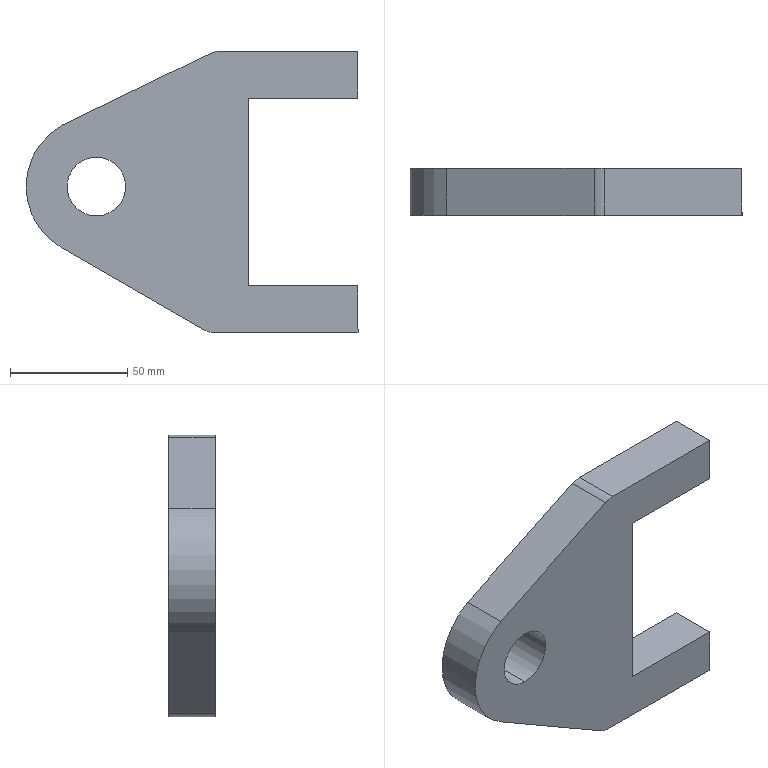Component | SolidWorks | 7TractionPlate-2 | 1 solid | 16 faces | box 141.51 x 20 x 120 mm | volume 186716 mm3 | plane 11 | cylinder 5 | commonest cylinder face diameters 25 x2 20 x2 60 x1
build123d program:
from build123d import *

# Parameters (mm, degrees)
SKETCH1_R           = 12.5
BOSS_EXTRUDE1_DEPTH = 20


with BuildPart() as part:
    # Sketch1 → Boss-Extrude1 (new body)
    with BuildSketch(Plane.XY):
        with BuildLine():
            Line((-34.563, 94.573), (-69.563, 33.951))
            ThreePointArc((-69.563, 33.951), (-70.562, 31.539), (-70.903, 28.951))
            Line((-70.903, 28.951), (-70.903, -31.936))
            Line((-70.903, -31.936), (-50.903, -31.936))
            Line((-50.903, -31.936), (-50.903, 14.622))
            Line((-50.903, 14.622), (29.097, 14.622))
            Line((29.097, 14.622), (29.097, -31.936))
            Line((29.097, -31.936), (40, -31.936))
            Line((40, -31.936), (49.097, -31.936))
            Line((49.097, -31.936), (49.097, 26.72))
            ThreePointArc((49.097, 26.72), (48.845, 28.95), (48.102, 31.068))
            Line((48.102, 31.068), (17.664, 94.104))
            ThreePointArc((17.664, 94.104), (-8.313, 109.571), (-34.563, 94.573))
        make_face()
        with Locations((-8.582, 79.573)):
            Circle(SKETCH1_R, mode=Mode.SUBTRACT)
    extrude(amount=BOSS_EXTRUDE1_DEPTH)


solid = part.part

# Placed as in the assembly
solid = solid.moved(Location((213.102, -253.79, 608.582), (90, 0, 90)))
STEP:
#1=COLOUR_RGB('',0.7922,0.8196,0.9333);
#2=FILL_AREA_STYLE_COLOUR('',#1);
#3=FILL_AREA_STYLE('',(#2));
#4=SURFACE_STYLE_FILL_AREA(#3);
#5=SURFACE_SIDE_STYLE('',(#4));
#6=SURFACE_STYLE_USAGE(.BOTH.,#5);
#7=PRESENTATION_STYLE_ASSIGNMENT((#6));
#8=CARTESIAN_POINT('',(5.257,-10.779,23.13));
#9=VERTEX_POINT('',#8);
#10=CARTESIAN_POINT('',(5.257,-10.779,24.114));
#11=VERTEX_POINT('',#10);
#12=CARTESIAN_POINT('',(5.257,-10.779,23.622));
#13=DIRECTION('',(0.,-1.,0.));
#14=DIRECTION('',(-0.,0.,1.));
#15=AXIS2_PLACEMENT_3D('',#12,#13,#14);
#16=CIRCLE('',#15,0.4921);
#17=EDGE_CURVE('',#9,#11,#16,.T.);
#18=ORIENTED_EDGE('',*,*,#17,.T.);
#19=CARTESIAN_POINT('',(5.257,-9.992,24.114));
#20=VERTEX_POINT('',#19);
#21=CARTESIAN_POINT('',(5.257,-10.779,24.114));
#22=DIRECTION('',(-0.,1.,-0.));
#23=VECTOR('',#22,39.37);
#24=LINE('',#21,#23);
#25=EDGE_CURVE('',#11,#20,#24,.T.);
#26=ORIENTED_EDGE('',*,*,#25,.T.);
#27=CARTESIAN_POINT('',(5.257,-9.992,23.13));
#28=VERTEX_POINT('',#27);
#29=CARTESIAN_POINT('',(5.257,-9.992,23.622));
#30=DIRECTION('',(0.,-1.,0.));
#31=DIRECTION('',(-0.,0.,1.));
#32=AXIS2_PLACEMENT_3D('',#29,#30,#31);
#33=CIRCLE('',#32,0.4921);
#34=EDGE_CURVE('',#28,#20,#33,.T.);
#35=ORIENTED_EDGE('',*,*,#34,.F.);
#36=CARTESIAN_POINT('',(5.257,-10.779,23.13));
#37=DIRECTION('',(-0.,1.,-0.));
#38=VECTOR('',#37,39.37);
#39=LINE('',#36,#38);
#40=EDGE_CURVE('',#9,#28,#39,.T.);
#41=ORIENTED_EDGE('',*,*,#40,.F.);
#42=EDGE_LOOP('',(#18,#26,#35,#41));
#43=FACE_OUTER_BOUND('',#42,.T.);
#44=CARTESIAN_POINT('',(5.257,-10.779,23.622));
#45=DIRECTION('',(-0.,1.,-0.));
#46=DIRECTION('',(0.,-0.,-1.));
#47=AXIS2_PLACEMENT_3D('',#44,#45,#46);
#48=CYLINDRICAL_SURFACE('',#47,0.4921);
#49=ADVANCED_FACE('',(#43),#48,.F.);
#50=CARTESIAN_POINT('',(7.25,-9.992,21.168));
#51=VERTEX_POINT('',#50);
#52=CARTESIAN_POINT('',(7.053,-9.992,21.221));
#53=VERTEX_POINT('',#52);
#54=CARTESIAN_POINT('',(7.25,-9.992,21.562));
#55=DIRECTION('',(-0.,1.,-0.));
#56=DIRECTION('',(-0.,0.,1.));
#57=AXIS2_PLACEMENT_3D('',#54,#55,#56);
#58=CIRCLE('',#57,0.3937);
#59=EDGE_CURVE('',#51,#53,#58,.T.);
#60=ORIENTED_EDGE('',*,*,#59,.F.);
#61=CARTESIAN_POINT('',(7.25,-10.779,21.168));
#62=VERTEX_POINT('',#61);
#63=CARTESIAN_POINT('',(7.25,-10.779,21.168));
#64=DIRECTION('',(-0.,1.,-0.));
#65=VECTOR('',#64,39.37);
#66=LINE('',#63,#65);
#67=EDGE_CURVE('',#62,#51,#66,.T.);
#68=ORIENTED_EDGE('',*,*,#67,.F.);
#69=CARTESIAN_POINT('',(7.053,-10.779,21.221));
#70=VERTEX_POINT('',#69);
#71=CARTESIAN_POINT('',(7.25,-10.779,21.562));
#72=DIRECTION('',(-0.,1.,-0.));
#73=DIRECTION('',(0.,0.,1.));
#74=AXIS2_PLACEMENT_3D('',#71,#72,#73);
#75=CIRCLE('',#74,0.3937);
#76=EDGE_CURVE('',#62,#70,#75,.T.);
#77=ORIENTED_EDGE('',*,*,#76,.T.);
#78=CARTESIAN_POINT('',(7.053,-10.779,21.221));
#79=DIRECTION('',(-0.,1.,-0.));
#80=VECTOR('',#79,39.37);
#81=LINE('',#78,#80);
#82=EDGE_CURVE('',#70,#53,#81,.T.);
#83=ORIENTED_EDGE('',*,*,#82,.T.);
#84=EDGE_LOOP('',(#60,#68,#77,#83));
#85=FACE_OUTER_BOUND('',#84,.T.);
#86=CARTESIAN_POINT('',(7.25,-10.779,21.562));
#87=DIRECTION('',(-0.,1.,-0.));
#88=DIRECTION('',(0.,-0.,-1.));
#89=AXIS2_PLACEMENT_3D('',#86,#87,#88);
#90=CYLINDRICAL_SURFACE('',#89,0.3937);
#91=ADVANCED_FACE('',(#85),#90,.T.);
#92=CARTESIAN_POINT('',(9.647,-9.992,21.168));
#93=VERTEX_POINT('',#92);
#94=CARTESIAN_POINT('',(8.39,-9.992,21.168));
#95=DIRECTION('',(1.,0.,0.));
#96=VECTOR('',#95,39.37);
#97=LINE('',#94,#96);
#98=EDGE_CURVE('',#51,#93,#97,.T.);
#99=ORIENTED_EDGE('',*,*,#98,.T.);
#100=CARTESIAN_POINT('',(9.647,-10.779,21.168));
#101=VERTEX_POINT('',#100);
#102=CARTESIAN_POINT('',(9.647,-10.779,21.168));
#103=DIRECTION('',(-0.,1.,-0.));
#104=VECTOR('',#103,39.37);
#105=LINE('',#102,#104);
#106=EDGE_CURVE('',#101,#93,#105,.T.);
#107=ORIENTED_EDGE('',*,*,#106,.F.);
#108=CARTESIAN_POINT('',(8.39,-10.779,21.168));
#109=DIRECTION('',(1.,0.,0.));
#110=VECTOR('',#109,39.37);
#111=LINE('',#108,#110);
#112=EDGE_CURVE('',#62,#101,#111,.T.);
#113=ORIENTED_EDGE('',*,*,#112,.F.);
#114=ORIENTED_EDGE('',*,*,#67,.T.);
#115=EDGE_LOOP('',(#99,#107,#113,#114));
#116=FACE_OUTER_BOUND('',#115,.T.);
#117=CARTESIAN_POINT('',(8.39,-10.779,21.168));
#118=DIRECTION('',(-0.,0.,1.));
#119=DIRECTION('',(-1.,-0.,-0.));
#120=AXIS2_PLACEMENT_3D('',#117,#118,#119);
#121=PLANE('',#120);
#122=ADVANCED_FACE('',(#116),#121,.F.);
#123=CARTESIAN_POINT('',(9.647,-9.992,21.956));
#124=VERTEX_POINT('',#123);
#125=CARTESIAN_POINT('',(9.647,-9.992,23.96));
#126=DIRECTION('',(-0.,0.,1.));
#127=VECTOR('',#126,39.37);
#128=LINE('',#125,#127);
#129=EDGE_CURVE('',#93,#124,#128,.T.);
#130=ORIENTED_EDGE('',*,*,#129,.T.);
#131=CARTESIAN_POINT('',(9.647,-10.779,21.956));
#132=VERTEX_POINT('',#131);
#133=CARTESIAN_POINT('',(9.647,-10.779,21.956));
#134=DIRECTION('',(-0.,1.,-0.));
#135=VECTOR('',#134,39.37);
#136=LINE('',#133,#135);
#137=EDGE_CURVE('',#132,#124,#136,.T.);
#138=ORIENTED_EDGE('',*,*,#137,.F.);
#139=CARTESIAN_POINT('',(9.647,-10.779,23.96));
#140=DIRECTION('',(-0.,0.,1.));
#141=VECTOR('',#140,39.37);
#142=LINE('',#139,#141);
#143=EDGE_CURVE('',#101,#132,#142,.T.);
#144=ORIENTED_EDGE('',*,*,#143,.F.);
#145=ORIENTED_EDGE('',*,*,#106,.T.);
#146=EDGE_LOOP('',(#130,#138,#144,#145));
#147=FACE_OUTER_BOUND('',#146,.T.);
#148=CARTESIAN_POINT('',(9.647,-10.779,23.96));
#149=DIRECTION('',(-1.,-0.,-0.));
#150=DIRECTION('',(0.,-1.,0.));
#151=AXIS2_PLACEMENT_3D('',#148,#149,#150);
#152=PLANE('',#151);
#153=ADVANCED_FACE('',(#147),#152,.F.);
#154=CARTESIAN_POINT('',(7.814,-9.992,21.956));
#155=VERTEX_POINT('',#154);
#156=CARTESIAN_POINT('',(8.39,-9.992,21.956));
#157=DIRECTION('',(-1.,-0.,-0.));
#158=VECTOR('',#157,39.37);
#159=LINE('',#156,#158);
#160=EDGE_CURVE('',#124,#155,#159,.T.);
#161=ORIENTED_EDGE('',*,*,#160,.T.);
#162=CARTESIAN_POINT('',(7.814,-10.779,21.956));
#163=VERTEX_POINT('',#162);
#164=CARTESIAN_POINT('',(7.814,-10.779,21.956));
#165=DIRECTION('',(-0.,1.,-0.));
#166=VECTOR('',#165,39.37);
#167=LINE('',#164,#166);
#168=EDGE_CURVE('',#163,#155,#167,.T.);
#169=ORIENTED_EDGE('',*,*,#168,.F.);
#170=CARTESIAN_POINT('',(8.39,-10.779,21.956));
#171=DIRECTION('',(-1.,-0.,-0.));
#172=VECTOR('',#171,39.37);
#173=LINE('',#170,#172);
#174=EDGE_CURVE('',#132,#163,#173,.T.);
#175=ORIENTED_EDGE('',*,*,#174,.F.);
#176=ORIENTED_EDGE('',*,*,#137,.T.);
#177=EDGE_LOOP('',(#161,#169,#175,#176));
#178=FACE_OUTER_BOUND('',#177,.T.);
#179=CARTESIAN_POINT('',(8.39,-10.779,21.956));
#180=DIRECTION('',(0.,-0.,-1.));
#181=DIRECTION('',(0.,-1.,0.));
#182=AXIS2_PLACEMENT_3D('',#179,#180,#181);
#183=PLANE('',#182);
#184=ADVANCED_FACE('',(#178),#183,.F.);
#185=CARTESIAN_POINT('',(7.814,-9.992,25.105));
#186=VERTEX_POINT('',#185);
#187=CARTESIAN_POINT('',(7.814,-9.992,23.96));
#188=DIRECTION('',(-0.,0.,1.));
#189=VECTOR('',#188,39.37);
#190=LINE('',#187,#189);
#191=EDGE_CURVE('',#155,#186,#190,.T.);
#192=ORIENTED_EDGE('',*,*,#191,.T.);
#193=CARTESIAN_POINT('',(7.814,-10.779,25.105));
#194=VERTEX_POINT('',#193);
#195=CARTESIAN_POINT('',(7.814,-10.779,25.105));
#196=DIRECTION('',(-0.,1.,-0.));
#197=VECTOR('',#196,39.37);
#198=LINE('',#195,#197);
#199=EDGE_CURVE('',#194,#186,#198,.T.);
#200=ORIENTED_EDGE('',*,*,#199,.F.);
#201=CARTESIAN_POINT('',(7.814,-10.779,23.96));
#202=DIRECTION('',(-0.,0.,1.));
#203=VECTOR('',#202,39.37);
#204=LINE('',#201,#203);
#205=EDGE_CURVE('',#163,#194,#204,.T.);
#206=ORIENTED_EDGE('',*,*,#205,.F.);
#207=ORIENTED_EDGE('',*,*,#168,.T.);
#208=EDGE_LOOP('',(#192,#200,#206,#207));
#209=FACE_OUTER_BOUND('',#208,.T.);
#210=CARTESIAN_POINT('',(7.814,-10.779,23.96));
#211=DIRECTION('',(-1.,-0.,-0.));
#212=DIRECTION('',(0.,-1.,0.));
#213=AXIS2_PLACEMENT_3D('',#210,#211,#212);
#214=PLANE('',#213);
#215=ADVANCED_FACE('',(#209),#214,.F.);
#216=CARTESIAN_POINT('',(9.647,-9.992,25.105));
#217=VERTEX_POINT('',#216);
#218=CARTESIAN_POINT('',(8.39,-9.992,25.105));
#219=DIRECTION('',(1.,0.,0.));
#220=VECTOR('',#219,39.37);
#221=LINE('',#218,#220);
#222=EDGE_CURVE('',#186,#217,#221,.T.);
#223=ORIENTED_EDGE('',*,*,#222,.T.);
#224=CARTESIAN_POINT('',(9.647,-10.779,25.105));
#225=VERTEX_POINT('',#224);
#226=CARTESIAN_POINT('',(9.647,-10.779,25.105));
#227=DIRECTION('',(-0.,1.,-0.));
#228=VECTOR('',#227,39.37);
#229=LINE('',#226,#228);
#230=EDGE_CURVE('',#225,#217,#229,.T.);
#231=ORIENTED_EDGE('',*,*,#230,.F.);
#232=CARTESIAN_POINT('',(8.39,-10.779,25.105));
#233=DIRECTION('',(1.,0.,0.));
#234=VECTOR('',#233,39.37);
#235=LINE('',#232,#234);
#236=EDGE_CURVE('',#194,#225,#235,.T.);
#237=ORIENTED_EDGE('',*,*,#236,.F.);
#238=ORIENTED_EDGE('',*,*,#199,.T.);
#239=EDGE_LOOP('',(#223,#231,#237,#238));
#240=FACE_OUTER_BOUND('',#239,.T.);
#241=CARTESIAN_POINT('',(8.39,-10.779,25.105));
#242=DIRECTION('',(-0.,0.,1.));
#243=DIRECTION('',(-0.,1.,-0.));
#244=AXIS2_PLACEMENT_3D('',#241,#242,#243);
#245=PLANE('',#244);
#246=ADVANCED_FACE('',(#240),#245,.F.);
#247=CARTESIAN_POINT('',(9.647,-9.992,25.893));
#248=VERTEX_POINT('',#247);
#249=CARTESIAN_POINT('',(9.647,-9.992,23.96));
#250=DIRECTION('',(-0.,0.,1.));
#251=VECTOR('',#250,39.37);
#252=LINE('',#249,#251);
#253=EDGE_CURVE('',#217,#248,#252,.T.);
#254=ORIENTED_EDGE('',*,*,#253,.T.);
#255=CARTESIAN_POINT('',(9.647,-10.779,25.893));
#256=VERTEX_POINT('',#255);
#257=CARTESIAN_POINT('',(9.647,-10.779,25.893));
#258=DIRECTION('',(-0.,1.,-0.));
#259=VECTOR('',#258,39.37);
#260=LINE('',#257,#259);
#261=EDGE_CURVE('',#256,#248,#260,.T.);
#262=ORIENTED_EDGE('',*,*,#261,.F.);
#263=CARTESIAN_POINT('',(9.647,-10.779,23.96));
#264=DIRECTION('',(-0.,0.,1.));
#265=VECTOR('',#264,39.37);
#266=LINE('',#263,#265);
#267=EDGE_CURVE('',#225,#256,#266,.T.);
#268=ORIENTED_EDGE('',*,*,#267,.F.);
#269=ORIENTED_EDGE('',*,*,#230,.T.);
#270=EDGE_LOOP('',(#254,#262,#268,#269));
#271=FACE_OUTER_BOUND('',#270,.T.);
#272=CARTESIAN_POINT('',(9.647,-10.779,23.96));
#273=DIRECTION('',(-1.,-0.,-0.));
#274=DIRECTION('',(0.,-0.,-1.));
#275=AXIS2_PLACEMENT_3D('',#272,#273,#274);
#276=PLANE('',#275);
#277=ADVANCED_FACE('',(#271),#276,.F.);
#278=CARTESIAN_POINT('',(7.338,-9.992,25.893));
#279=VERTEX_POINT('',#278);
#280=CARTESIAN_POINT('',(8.39,-9.992,25.893));
#281=DIRECTION('',(1.,0.,0.));
#282=VECTOR('',#281,39.37);
#283=LINE('',#280,#282);
#284=EDGE_CURVE('',#279,#248,#283,.T.);
#285=ORIENTED_EDGE('',*,*,#284,.F.);
#286=CARTESIAN_POINT('',(7.338,-10.779,25.893));
#287=VERTEX_POINT('',#286);
#288=CARTESIAN_POINT('',(7.338,-10.779,25.893));
#289=DIRECTION('',(-0.,1.,-0.));
#290=VECTOR('',#289,39.37);
#291=LINE('',#288,#290);
#292=EDGE_CURVE('',#287,#279,#291,.T.);
#293=ORIENTED_EDGE('',*,*,#292,.F.);
#294=CARTESIAN_POINT('',(8.39,-10.779,25.893));
#295=DIRECTION('',(1.,0.,0.));
#296=VECTOR('',#295,39.37);
#297=LINE('',#294,#296);
#298=EDGE_CURVE('',#287,#256,#297,.T.);
#299=ORIENTED_EDGE('',*,*,#298,.T.);
#300=ORIENTED_EDGE('',*,*,#261,.T.);
#301=EDGE_LOOP('',(#285,#293,#299,#300));
#302=FACE_OUTER_BOUND('',#301,.T.);
#303=CARTESIAN_POINT('',(8.39,-10.779,25.893));
#304=DIRECTION('',(-0.,0.,1.));
#305=DIRECTION('',(-1.,-0.,-0.));
#306=AXIS2_PLACEMENT_3D('',#303,#304,#305);
#307=PLANE('',#306);
#308=ADVANCED_FACE('',(#302),#307,.T.);
#309=CARTESIAN_POINT('',(7.167,-9.992,25.854));
#310=VERTEX_POINT('',#309);
#311=CARTESIAN_POINT('',(7.338,-9.992,25.499));
#312=DIRECTION('',(0.,-1.,0.));
#313=DIRECTION('',(-0.,0.,1.));
#314=AXIS2_PLACEMENT_3D('',#311,#312,#313);
#315=CIRCLE('',#314,0.3937);
#316=EDGE_CURVE('',#279,#310,#315,.T.);
#317=ORIENTED_EDGE('',*,*,#316,.T.);
#318=CARTESIAN_POINT('',(7.167,-10.779,25.854));
#319=VERTEX_POINT('',#318);
#320=CARTESIAN_POINT('',(7.167,-10.779,25.854));
#321=DIRECTION('',(-0.,1.,-0.));
#322=VECTOR('',#321,39.37);
#323=LINE('',#320,#322);
#324=EDGE_CURVE('',#319,#310,#323,.T.);
#325=ORIENTED_EDGE('',*,*,#324,.F.);
#326=CARTESIAN_POINT('',(7.338,-10.779,25.499));
#327=DIRECTION('',(0.,-1.,0.));
#328=DIRECTION('',(-0.,0.,1.));
#329=AXIS2_PLACEMENT_3D('',#326,#327,#328);
#330=CIRCLE('',#329,0.3937);
#331=EDGE_CURVE('',#287,#319,#330,.T.);
#332=ORIENTED_EDGE('',*,*,#331,.F.);
#333=ORIENTED_EDGE('',*,*,#292,.T.);
#334=EDGE_LOOP('',(#317,#325,#332,#333));
#335=FACE_OUTER_BOUND('',#334,.T.);
#336=CARTESIAN_POINT('',(7.338,-10.779,25.499));
#337=DIRECTION('',(-0.,1.,-0.));
#338=DIRECTION('',(0.,-0.,-1.));
#339=AXIS2_PLACEMENT_3D('',#336,#337,#338);
#340=CYLINDRICAL_SURFACE('',#339,0.3937);
#341=ADVANCED_FACE('',(#335),#340,.T.);
#342=CARTESIAN_POINT('',(4.685,-9.992,24.655));
#343=VERTEX_POINT('',#342);
#344=CARTESIAN_POINT('',(7.417,-9.992,25.975));
#345=DIRECTION('',(0.9005,0.,0.4348));
#346=VECTOR('',#345,39.37);
#347=LINE('',#344,#346);
#348=EDGE_CURVE('',#343,#310,#347,.T.);
#349=ORIENTED_EDGE('',*,*,#348,.F.);
#350=CARTESIAN_POINT('',(4.685,-10.779,24.655));
#351=VERTEX_POINT('',#350);
#352=CARTESIAN_POINT('',(4.685,-10.779,24.655));
#353=DIRECTION('',(-0.,1.,-0.));
#354=VECTOR('',#353,39.37);
#355=LINE('',#352,#354);
#356=EDGE_CURVE('',#351,#343,#355,.T.);
#357=ORIENTED_EDGE('',*,*,#356,.F.);
#358=CARTESIAN_POINT('',(7.417,-10.779,25.975));
#359=DIRECTION('',(0.9005,0.,0.4348));
#360=VECTOR('',#359,39.37);
#361=LINE('',#358,#360);
#362=EDGE_CURVE('',#351,#319,#361,.T.);
#363=ORIENTED_EDGE('',*,*,#362,.T.);
#364=ORIENTED_EDGE('',*,*,#324,.T.);
#365=EDGE_LOOP('',(#349,#357,#363,#364));
#366=FACE_OUTER_BOUND('',#365,.T.);
#367=CARTESIAN_POINT('',(7.417,-10.779,25.975));
#368=DIRECTION('',(-0.4348,0.,0.9005));
#369=DIRECTION('',(-0.9005,-0.,-0.4348));
#370=AXIS2_PLACEMENT_3D('',#367,#368,#369);
#371=PLANE('',#370);
#372=ADVANCED_FACE('',(#366),#371,.T.);
#373=CARTESIAN_POINT('',(4.667,-9.992,22.599));
#374=VERTEX_POINT('',#373);
#375=CARTESIAN_POINT('',(5.257,-9.992,23.622));
#376=DIRECTION('',(-0.,1.,-0.));
#377=DIRECTION('',(-0.,0.,1.));
#378=AXIS2_PLACEMENT_3D('',#375,#376,#377);
#379=CIRCLE('',#378,1.181);
#380=EDGE_CURVE('',#374,#343,#379,.T.);
#381=ORIENTED_EDGE('',*,*,#380,.F.);
#382=CARTESIAN_POINT('',(4.667,-10.779,22.599));
#383=VERTEX_POINT('',#382);
#384=CARTESIAN_POINT('',(4.667,-10.779,22.599));
#385=DIRECTION('',(-0.,1.,-0.));
#386=VECTOR('',#385,39.37);
#387=LINE('',#384,#386);
#388=EDGE_CURVE('',#383,#374,#387,.T.);
#389=ORIENTED_EDGE('',*,*,#388,.F.);
#390=CARTESIAN_POINT('',(5.257,-10.779,23.622));
#391=DIRECTION('',(-0.,1.,-0.));
#392=DIRECTION('',(-0.,0.,1.));
#393=AXIS2_PLACEMENT_3D('',#390,#391,#392);
#394=CIRCLE('',#393,1.181);
#395=EDGE_CURVE('',#383,#351,#394,.T.);
#396=ORIENTED_EDGE('',*,*,#395,.T.);
#397=ORIENTED_EDGE('',*,*,#356,.T.);
#398=EDGE_LOOP('',(#381,#389,#396,#397));
#399=FACE_OUTER_BOUND('',#398,.T.);
#400=CARTESIAN_POINT('',(5.257,-10.779,23.622));
#401=DIRECTION('',(-0.,1.,-0.));
#402=DIRECTION('',(0.,-0.,-1.));
#403=AXIS2_PLACEMENT_3D('',#400,#401,#402);
#404=CYLINDRICAL_SURFACE('',#403,1.181);
#405=ADVANCED_FACE('',(#399),#404,.T.);
#406=ORIENTED_EDGE('',*,*,#25,.F.);
#407=CARTESIAN_POINT('',(5.257,-10.779,23.622));
#408=DIRECTION('',(0.,-1.,0.));
#409=DIRECTION('',(-0.,0.,1.));
#410=AXIS2_PLACEMENT_3D('',#407,#408,#409);
#411=CIRCLE('',#410,0.4921);
#412=EDGE_CURVE('',#11,#9,#411,.T.);
#413=ORIENTED_EDGE('',*,*,#412,.T.);
#414=ORIENTED_EDGE('',*,*,#40,.T.);
#415=CARTESIAN_POINT('',(5.257,-9.992,23.622));
#416=DIRECTION('',(0.,-1.,0.));
#417=DIRECTION('',(-0.,0.,1.));
#418=AXIS2_PLACEMENT_3D('',#415,#416,#417);
#419=CIRCLE('',#418,0.4921);
#420=EDGE_CURVE('',#20,#28,#419,.T.);
#421=ORIENTED_EDGE('',*,*,#420,.F.);
#422=EDGE_LOOP('',(#406,#413,#414,#421));
#423=FACE_OUTER_BOUND('',#422,.T.);
#424=CARTESIAN_POINT('',(5.257,-10.779,23.622));
#425=DIRECTION('',(-0.,1.,-0.));
#426=DIRECTION('',(0.,-0.,-1.));
#427=AXIS2_PLACEMENT_3D('',#424,#425,#426);
#428=CYLINDRICAL_SURFACE('',#427,0.4921);
#429=ADVANCED_FACE('',(#423),#428,.F.);
#430=CARTESIAN_POINT('',(6.87,-9.992,21.327));
#431=DIRECTION('',(-0.866,-0.,0.5));
#432=VECTOR('',#431,39.37);
#433=LINE('',#430,#432);
#434=EDGE_CURVE('',#53,#374,#433,.T.);
#435=ORIENTED_EDGE('',*,*,#434,.F.);
#436=ORIENTED_EDGE('',*,*,#82,.F.);
#437=CARTESIAN_POINT('',(6.87,-10.779,21.327));
#438=DIRECTION('',(-0.866,-0.,0.5));
#439=VECTOR('',#438,39.37);
#440=LINE('',#437,#439);
#441=EDGE_CURVE('',#70,#383,#440,.T.);
#442=ORIENTED_EDGE('',*,*,#441,.T.);
#443=ORIENTED_EDGE('',*,*,#388,.T.);
#444=EDGE_LOOP('',(#435,#436,#442,#443));
#445=FACE_OUTER_BOUND('',#444,.T.);
#446=CARTESIAN_POINT('',(6.87,-10.779,21.327));
#447=DIRECTION('',(-0.5,-0.,-0.866));
#448=DIRECTION('',(0.866,0.,-0.5));
#449=AXIS2_PLACEMENT_3D('',#446,#447,#448);
#450=PLANE('',#449);
#451=ADVANCED_FACE('',(#445),#450,.T.);
#452=ORIENTED_EDGE('',*,*,#17,.F.);
#453=ORIENTED_EDGE('',*,*,#412,.F.);
#454=EDGE_LOOP('',(#452,#453));
#455=FACE_BOUND('',#454,.T.);
#456=ORIENTED_EDGE('',*,*,#76,.F.);
#457=ORIENTED_EDGE('',*,*,#112,.T.);
#458=ORIENTED_EDGE('',*,*,#143,.T.);
#459=ORIENTED_EDGE('',*,*,#174,.T.);
#460=ORIENTED_EDGE('',*,*,#205,.T.);
#461=ORIENTED_EDGE('',*,*,#236,.T.);
#462=ORIENTED_EDGE('',*,*,#267,.T.);
#463=ORIENTED_EDGE('',*,*,#298,.F.);
#464=ORIENTED_EDGE('',*,*,#331,.T.);
#465=ORIENTED_EDGE('',*,*,#362,.F.);
#466=ORIENTED_EDGE('',*,*,#395,.F.);
#467=ORIENTED_EDGE('',*,*,#441,.F.);
#468=EDGE_LOOP('',(#456,#457,#458,#459,#460,#461,#462,#463,#464,#465,#466,#467));
#469=FACE_OUTER_BOUND('',#468,.T.);
#470=CARTESIAN_POINT('',(8.39,-10.779,23.96));
#471=DIRECTION('',(0.,-1.,0.));
#472=DIRECTION('',(-0.,0.,1.));
#473=AXIS2_PLACEMENT_3D('',#470,#471,#472);
#474=PLANE('',#473);
#475=ADVANCED_FACE('',(#455,#469),#474,.T.);
#476=ORIENTED_EDGE('',*,*,#34,.T.);
#477=ORIENTED_EDGE('',*,*,#420,.T.);
#478=EDGE_LOOP('',(#476,#477));
#479=FACE_BOUND('',#478,.T.);
#480=ORIENTED_EDGE('',*,*,#59,.T.);
#481=ORIENTED_EDGE('',*,*,#434,.T.);
#482=ORIENTED_EDGE('',*,*,#380,.T.);
#483=ORIENTED_EDGE('',*,*,#348,.T.);
#484=ORIENTED_EDGE('',*,*,#316,.F.);
#485=ORIENTED_EDGE('',*,*,#284,.T.);
#486=ORIENTED_EDGE('',*,*,#253,.F.);
#487=ORIENTED_EDGE('',*,*,#222,.F.);
#488=ORIENTED_EDGE('',*,*,#191,.F.);
#489=ORIENTED_EDGE('',*,*,#160,.F.);
#490=ORIENTED_EDGE('',*,*,#129,.F.);
#491=ORIENTED_EDGE('',*,*,#98,.F.);
#492=EDGE_LOOP('',(#480,#481,#482,#483,#484,#485,#486,#487,#488,#489,#490,#491));
#493=FACE_OUTER_BOUND('',#492,.T.);
#494=CARTESIAN_POINT('',(8.39,-9.992,23.96));
#495=DIRECTION('',(0.,-1.,0.));
#496=DIRECTION('',(-0.,0.,1.));
#497=AXIS2_PLACEMENT_3D('',#494,#495,#496);
#498=PLANE('',#497);
#499=ADVANCED_FACE('',(#479,#493),#498,.F.);
#500=CLOSED_SHELL('',(#49,#91,#122,#153,#184,#215,#246,#277,#308,#341,#372,#405,#429,#451,#475,#499));
#501=MANIFOLD_SOLID_BREP('',#500);
#502=STYLED_ITEM('',(#7),#501);
#503=(LENGTH_UNIT()NAMED_UNIT(*)SI_UNIT($,.METRE.));
#504=LENGTH_MEASURE_WITH_UNIT(LENGTH_MEASURE(0.0254),#503);
#505=DIMENSIONAL_EXPONENTS(1.,0.,0.,0.,0.,0.,0.);
#506=(CONVERSION_BASED_UNIT('',#504)LENGTH_UNIT()NAMED_UNIT(#505));
#507=UNCERTAINTY_MEASURE_WITH_UNIT(LENGTH_MEASURE(0.00001),#506,'','');
#508=(NAMED_UNIT(*)PLANE_ANGLE_UNIT()SI_UNIT($,.RADIAN.));
#509=(NAMED_UNIT(*)SI_UNIT($,.STERADIAN.)SOLID_ANGLE_UNIT());
#510=(GEOMETRIC_REPRESENTATION_CONTEXT(3)GLOBAL_UNCERTAINTY_ASSIGNED_CONTEXT((#507))GLOBAL_UNIT_ASSIGNED_CONTEXT((#506,#508,#509))REPRESENTATION_CONTEXT('',''));
#511=MECHANICAL_DESIGN_GEOMETRIC_PRESENTATION_REPRESENTATION('',(#502),#510);
#512=PRESENTATION_LAYER_ASSIGNMENT('','',(#502));
#513=CARTESIAN_POINT('',(0.,0.,0.));
#514=DIRECTION('',(0.,0.,1.));
#515=DIRECTION('',(1.,0.,0.));
#516=AXIS2_PLACEMENT_3D('',#513,#514,#515);
#517=(LENGTH_UNIT()NAMED_UNIT(*)SI_UNIT($,.METRE.));
#518=LENGTH_MEASURE_WITH_UNIT(LENGTH_MEASURE(0.0254),#517);
#519=DIMENSIONAL_EXPONENTS(1.,0.,0.,0.,0.,0.,0.);
#520=(CONVERSION_BASED_UNIT('',#518)LENGTH_UNIT()NAMED_UNIT(#519));
#521=UNCERTAINTY_MEASURE_WITH_UNIT(LENGTH_MEASURE(0.00001),#520,'','');
#522=(NAMED_UNIT(*)PLANE_ANGLE_UNIT()SI_UNIT($,.RADIAN.));
#523=(NAMED_UNIT(*)SI_UNIT($,.STERADIAN.)SOLID_ANGLE_UNIT());
#524=(GEOMETRIC_REPRESENTATION_CONTEXT(3)GLOBAL_UNCERTAINTY_ASSIGNED_CONTEXT((#521))GLOBAL_UNIT_ASSIGNED_CONTEXT((#520,#522,#523))REPRESENTATION_CONTEXT('',''));
#525=ADVANCED_BREP_SHAPE_REPRESENTATION('',(#501,#516),#524);